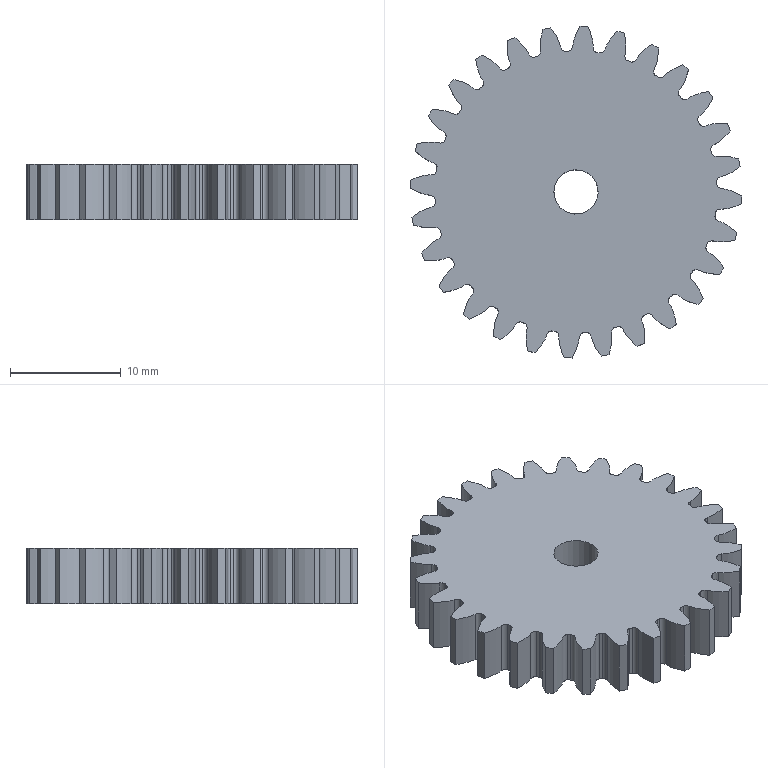Component | NX | GEAR_3 | 1 solid | 171 faces | volume 2974 mm3 | spline 140 | cylinder 29 | plane 2 | commonest cylinder face diameters 25.48 x28 4 x1